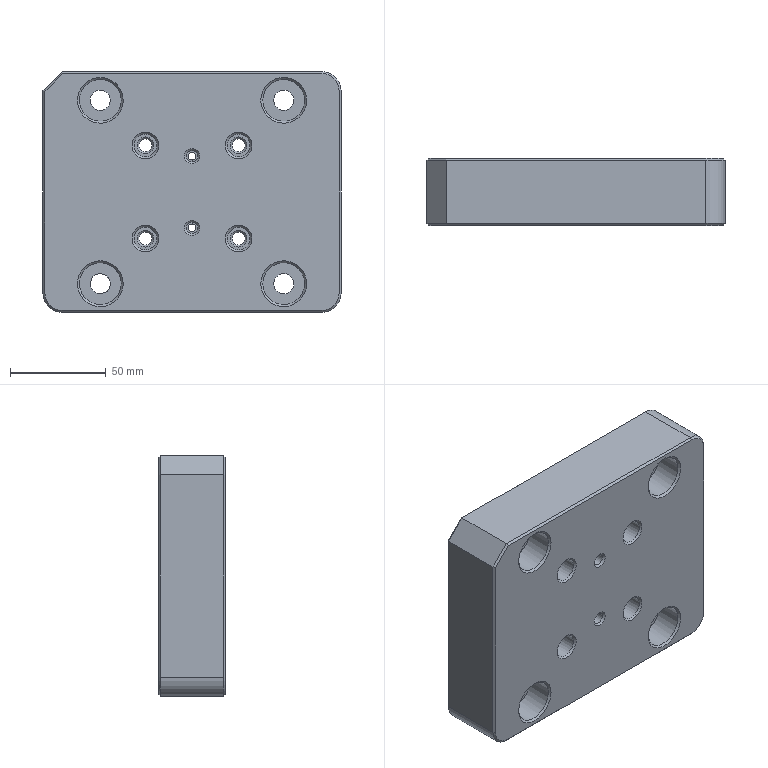CAM job | NX | mm | 3-axis | 5 set-ups | 54 operations | part box 156 x 35 x 126
set-up 1
1. Planar Roughing | Mill Mill5 LX-D12 | PLANAR_ROUGHING_1 | path 12004.66 mm | 2.914 min
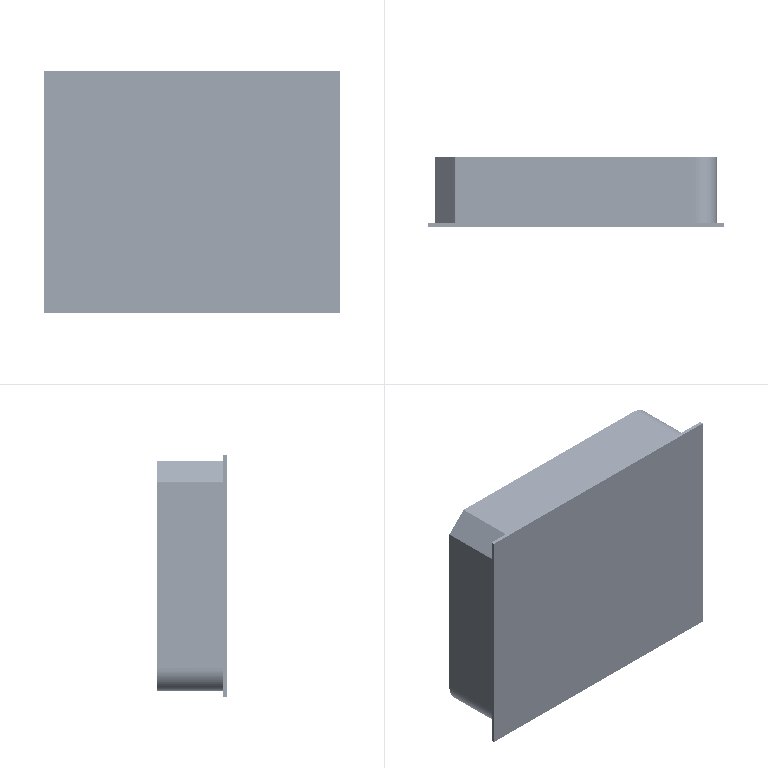2. Drilling | Mill MillChamfer DXZ-D10A90 | DRILLING_2 | path 180 mm | 0.0972 min
3. Drilling | Mill MillChamfer DXZ-D10A90 | DRILLING_3 | path 180 mm | 0.0972 min
4. Drilling | Drill DrillStandard ZT-D5.5 | DRILLING_4 | path 2708.533 mm | 3.216 min
5. Cylinder Milling | Mill Mill5 LX-D8 | CYLINDER_MILLING_5 | path 481.27 mm | 0.7684 min
6. Cylinder Milling | Mill Mill5 LX-D8 | CYLINDER_MILLING_6 | path 481.27 mm | 0.7684 min
7. Volume Based 2.5D Milling | Mill Mill5 LX-D8 | VOLUME_BASED_2.5D_MILLING_7 | path 6122.779 mm | 1.864 min
8. Planar Milling | Mill Mill5 LX-D12J | PLANAR_MILLING_8 | path 5705.557 mm | 2.835 min
set-up 2
9. Cylinder Milling | Mill Mill5 LX-D10 | CYLINDER_MILLING_9 | path 1152.137 mm | 1.219 min
10. Cylinder Milling | Mill Mill5 LX-D10 | CYLINDER_MILLING_10 | path 1152.137 mm | 1.219 min
11. Cylinder Milling | Mill Mill5 LX-D4 | CYLINDER_MILLING_11 | path 1233.176 mm | 1.159 min
12. Planar Milling | Mill Mill5 LX-D12J | PLANAR_MILLING_12 | path 2606.304 mm | 1.269 min
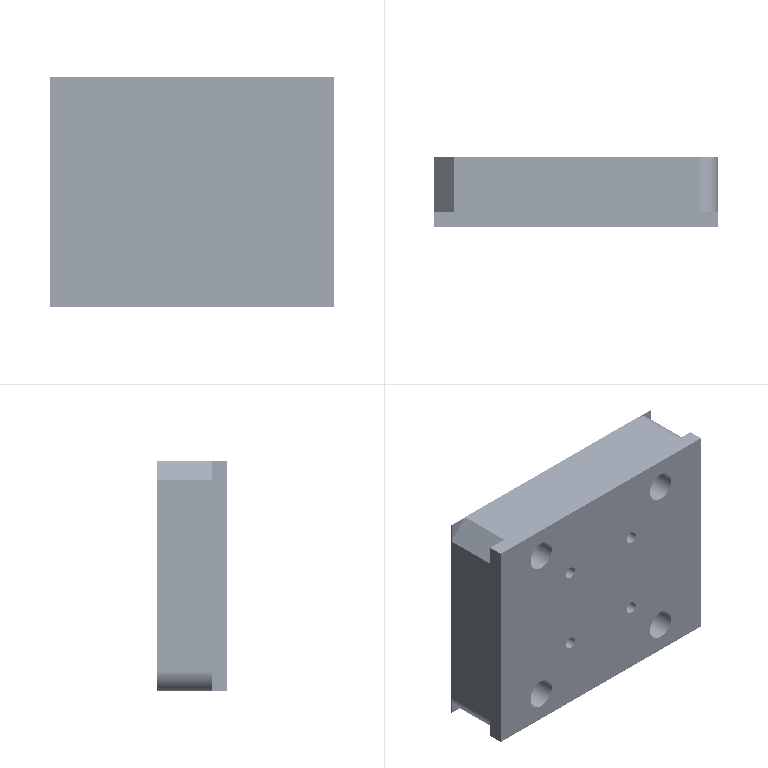set-up 3
13. Face Milling | Mill Mill5 E50R0.8 | FACE_MILLING_13 | path 3280.8 mm | 1.511 min
14. Planar Milling | Mill Mill5 LX-D12 | PLANAR_MILLING_14 | path 6543.772 mm | 1.583 min
15. Cavity Milling | Mill Mill5 LX-D12 | CAVITY_MILLING_15 | path 3066.563 mm | 0.8702 min
16. Cylinder Milling | Mill Mill5 LX-D10 | CYLINDER_MILLING_16 | path 1076.834 mm | 0.8077 min
17. Cylinder Milling | Mill Mill5 LX-D6 | CYLINDER_MILLING_17 | path 2028.479 mm | 1.894 min
18. Drilling | Mill MillChamfer DXZ-D6A90 | DRILLING_18 | path 334.371 mm | 0.1918 min
19. Drilling | Mill MillChamfer DXZ-D6A90 | DRILLING_19 | path 174.3 mm | 0.09663 min
20. Drilling | Drill DrillStandard ZT-D6.8 | DRILLING_20 | path 2132.603 mm | 2.755 min
21. Drilling | Drill DrillStandard ZT-D3.8 | DRILLING_21 | path 302 mm | 0.4423 min
22. Face Milling | Mill Mill5 E50R0.8 | FACE_MILLING_22 | path 1452.714 mm | 1.776 min
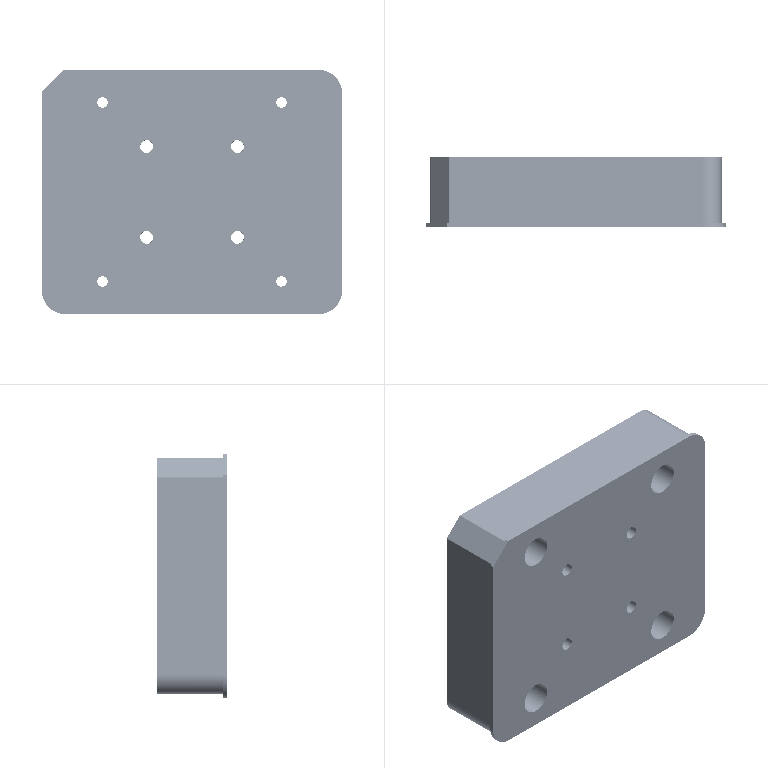23. Planar Milling | Mill Mill5 LX-D12J | PLANAR_MILLING_23 | path 1331.585 mm | 1.49 min
24. Volume Based 2.5D Milling | Mill Mill5 LX-D10J | VOLUME_BASED_2.5D_MILLING_24 | path 515.445 mm | 0.6478 min
25. Volume Based 2.5D Milling | Mill Mill5 LX-D10J | VOLUME_BASED_2.5D_MILLING_25 | path 196.595 mm | 0.1752 min
26. Cylinder Milling | Mill Mill5 LX-D10J | CYLINDER_MILLING_26 | path 1134.437 mm | 1.712 min
27. Cylinder Milling | Mill Mill5 LX-D6J | CYLINDER_MILLING_27 | path 1556.886 mm | 2.542 min
28. Cylinder Milling | Mill Mill5 LX-D3J | CYLINDER_MILLING_28 | path 377.826 mm | 0.5072 min
29. Volume Based 2.5D Milling | Mill MillChamfer DJ-D10A90 | VOLUME_BASED_2.5D_MILLING_29 | path 1611.25 mm | 1.004 min
30. Volume Based 2.5D Milling | Mill MillChamfer DJ-D10A90 | VOLUME_BASED_2.5D_MILLING_30 | path 618.624 mm | 0.5745 min
31. Volume Based 2.5D Milling | Mill MillChamfer DJ-D10A90 | VOLUME_BASED_2.5D_MILLING_31 | path 208.521 mm | 0.1644 min
32. Drilling | Mill MillChamfer DJ-D10A90 | DRILLING_32 | path 180.3 mm | 0.07663 min
33. Thread Milling | Drill DrillThreadMill M8X1.25-D6 | THREAD_MILLING_33 | path 2948.939 mm | 4.291 min
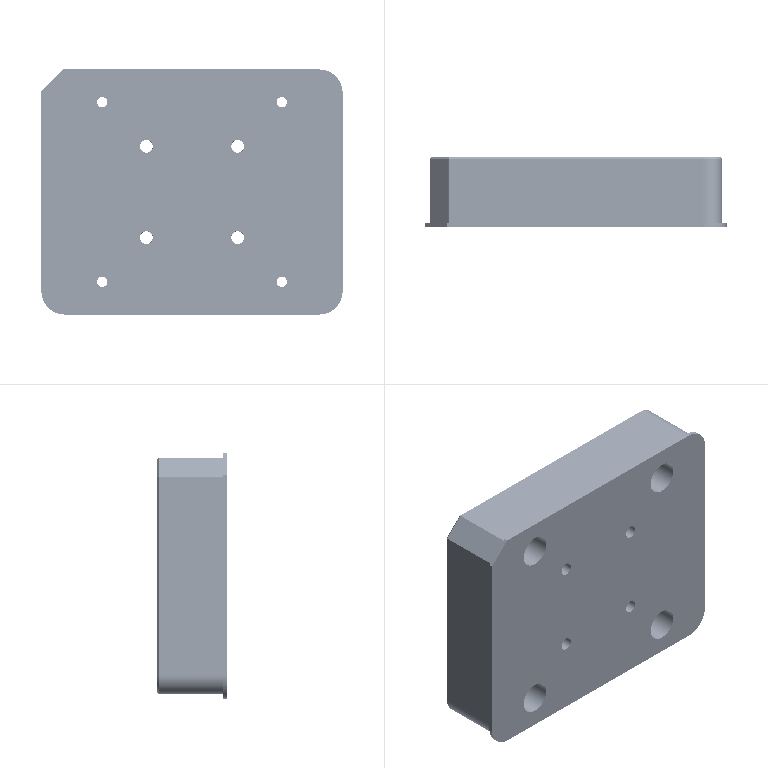34. Thread Milling | Drill DrillThreadMill M8X1.25-D6 | THREAD_MILLING_34 | path 967.738 mm | 1.133 min
35. Planar Milling | Mill Mill5 LX-D12J | PLANAR_MILLING_35 | path 6167.224 mm | 3.037 min
set-up 4
36. Face Milling | Mill Mill5 E50R0.8 | FACE_MILLING_36 | path 6664.5 mm | 3.032 min
37. Drilling | Mill MillChamfer DXZ-D10A90 | DRILLING_37 | path 121.5 mm | 0.09135 min
38. Drilling | Drill DrillStandard ZT-D5.0 | DRILLING_38 | path 372.7 mm | 0.7233 min
39. Cylinder Milling | Mill Mill5 LX-D12 | CYLINDER_MILLING_39 | path 4500.721 mm | 5.085 min
40. Cylinder Milling | Mill Mill5 LX-D8 | CYLINDER_MILLING_40 | path 1391.299 mm | 1.36 min
41. Cylinder Milling | Mill Mill5 LX-D4 | CYLINDER_MILLING_41 | path 522.297 mm | 0.4849 min
42. Face Milling | Mill Mill5 E50R0.8 | FACE_MILLING_42 | path 1461.714 mm | 1.777 min
43. Cylinder Milling | Mill Mill5 LX-D4J | CYLINDER_MILLING_43 | path 619.683 mm | 1.199 min
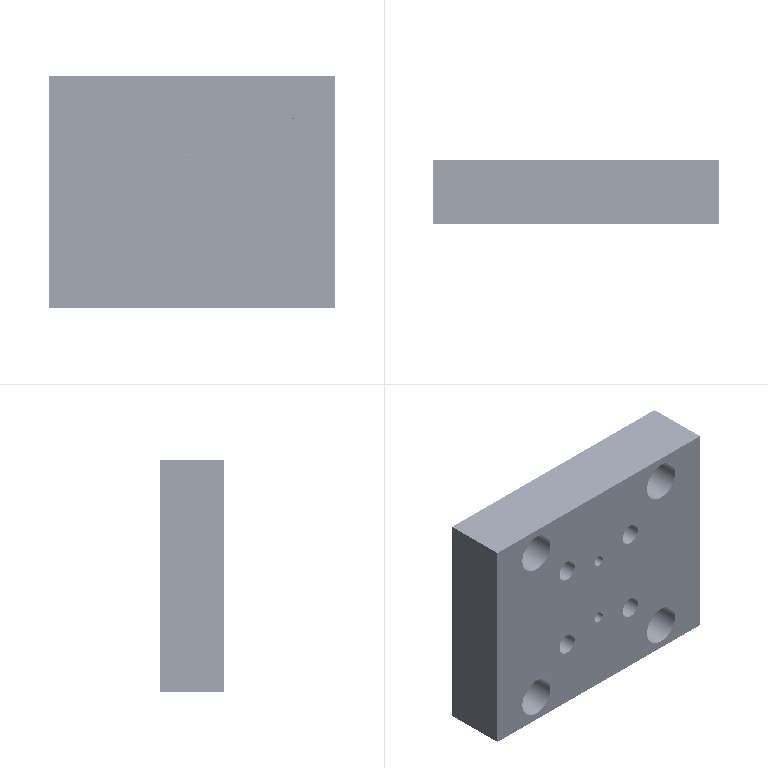44. Cylinder Milling | Mill Mill5 LX-D8J | CYLINDER_MILLING_44 | path 976.215 mm | 1.65 min
45. Cylinder Milling | Mill Mill5 LX-D12J | CYLINDER_MILLING_45 | path 2708.044 mm | 5.639 min
46. Volume Based 2.5D Milling | Mill MillChamfer DJ-D10A90 | VOLUME_BASED_2.5D_MILLING_46 | path 613.624 mm | 0.574 min
47. Volume Based 2.5D Milling | Mill MillChamfer DJ-D10A90 | VOLUME_BASED_2.5D_MILLING_47 | path 1789.297 mm | 1.902 min
48. Drilling | Mill MillChamfer DJ-D10A90 | DRILLING_48 | path 133.5 mm | 0.09125 min
49. Drilling | Mill MillChamfer DJ-D10A90 | DRILLING_49 | path 421.571 mm | 0.1498 min
50. Planar Milling | Mill Mill5 LX-D12 | PLANAR_MILLING_50 | path 706.361 mm | 0.7661 min
set-up 5
51. Z-Level Milling | Mill Mill5 LX-D10 | Z-LEVEL_MILLING_51 | path 1694.937 mm | 1.381 min
52. Z-Level Milling | Mill Mill5 LX-D10J | Z-LEVEL_MILLING_52 | path 511.161 mm | 0.7846 min
53. Planar Milling | Mill MillChamfer DJ-D6A90 | PLANAR_MILLING_53 | path 254.583 mm | 0.2764 min
54. Planar Text | Mill Mill5 KZ-D0.5R0.25 | PLANAR_TEXT_54 | path 11100.084 mm | 4.047 min